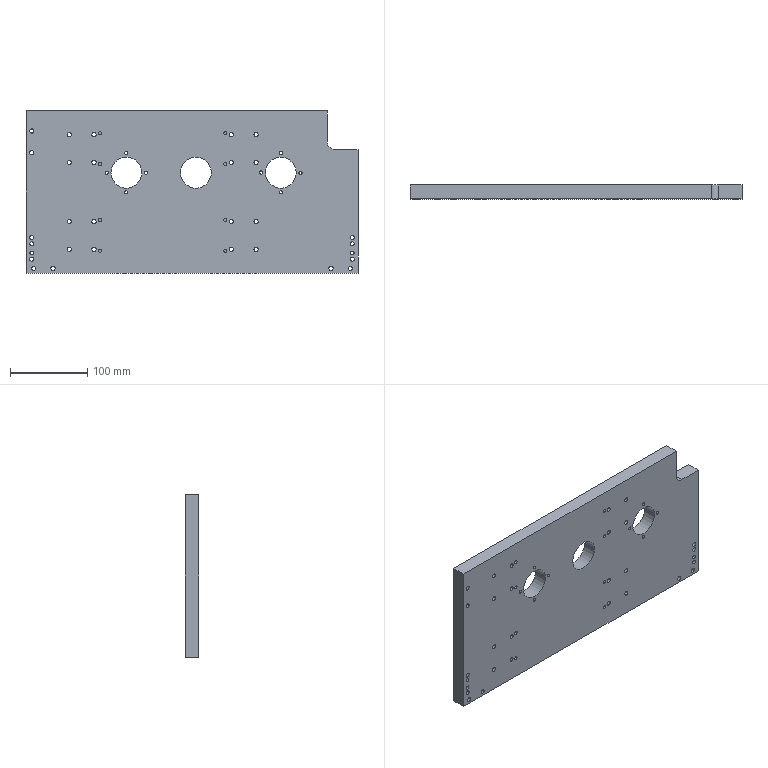Component | SolidWorks | PressingMechanism-06-1 | 1 solid | 193 faces | box 430 x 18 x 210 mm | volume 1498905 mm3 | cylinder 151 | plane 42 | commonest cylinder face diameters 10 x52 5.5 x52 4 x16 4.2 x16 5 x8 40 x6 20 x1
build123d program:
from build123d import *

# Parameters (mm, degrees)
SKETCH1_W                                           = 210
SKETCH1_H                                           = 480
EXTRUDE1_DEPTH                                      = 9
HOLEWZD1_D                                          = 40
MOVE_FACE1_BY                                       = 50
M5_TAPPED_HOLE1_D                                   = 4.2
CBORE_FOR_M5_HEX_SOCKET_HEAD_CAP_SCREW1_D           = 5.5
CBORE_FOR_M5_HEX_SOCKET_HEAD_CAP_SCREW1_CBORE_D     = 10
CBORE_FOR_M5_HEX_SOCKET_HEAD_CAP_SCREW1_CBORE_DEPTH = 5.4
HOLEWZD2_D                                          = 4
HOLEWZD2_DEPTH                                      = 8
CUT_EXTRUDE2_REACH                                  = 264.581
SKETCH14_W                                          = 50
SKETCH14_H                                          = 40
HOLEWZD3_D                                          = 5
CBORE_FOR_M5_HEX_SOCKET_HEAD_CAP_SCREW2_D           = 5.5
CBORE_FOR_M5_HEX_SOCKET_HEAD_CAP_SCREW2_CBORE_D     = 10
CBORE_FOR_M5_HEX_SOCKET_HEAD_CAP_SCREW2_CBORE_DEPTH = 5.4
FILLET1_R                                           = 10


with BuildPart() as part:
    # Sketch1 → Extrude1 (new, symmetric)
    with BuildSketch(Plane(origin=(0, 0, 0), x_dir=(1, 0, 0), z_dir=(0, 1, 0))):
        Rectangle(SKETCH1_W, SKETCH1_H)
    extrude(amount=EXTRUDE1_DEPTH, both=True)

    # HoleWzd1 (through all)
    with Locations(Plane(origin=(0, 9, 0), x_dir=(1, 0, 0), z_dir=(0, 1, 0))):
        with Locations((25, 30), (25, 140), (25, -60)):
            Hole(HOLEWZD1_D / 2)

    # Move Face1: a face moved inward by 50.0
    extrude(part.faces().sort_by_distance((0, 0, 240))[0], amount=MOVE_FACE1_BY, dir=(0, 0, -1), mode=Mode.SUBTRACT)

    # M5 Tapped Hole1 (through all)
    with Locations(Plane(origin=(0, 9, 0), x_dir=(1, 0, 0), z_dir=(0, 1, 0))):
        with Locations((25, -34.5), (-0.5, -60), (25, -85.5), (50.5, -60), (24.785, 165.499), (-0.4991, 139.785), (25.215, 114.501), (50.499, 140.215)):
            Hole(M5_TAPPED_HOLE1_D / 2)

    # CBORE for M5 Hex Socket Head Cap Screw1 (through all)
    with Locations(Plane(origin=(0, 9, 0), x_dir=(1, 0, 0), z_dir=(0, 1, 0))):
        with Locations((74.25, 108), (38.25, 108), (38.25, 76), (74.25, 76), (74.25, -102), (38.25, -102), (38.25, -134), (74.25, -134), (-74.25, -102), (-74.25, -134), (-38.25, -134), (-38.25, -102), (-74.25, 108), (-74.25, 76), (-38.25, 76), (-38.25, 108)):
            CounterBoreHole(CBORE_FOR_M5_HEX_SOCKET_HEAD_CAP_SCREW1_D / 2, CBORE_FOR_M5_HEX_SOCKET_HEAD_CAP_SCREW1_CBORE_D / 2, CBORE_FOR_M5_HEX_SOCKET_HEAD_CAP_SCREW1_CBORE_DEPTH)

    # HoleWzd2
    with Locations(Plane(origin=(0, -9, 0), x_dir=(-1, 0, 0), z_dir=(0, -1, 0))):
        with Locations((-76.25, 68), (-36.25, 68), (36.25, 68), (76.25, 68), (36.25, -94), (76.25, -94), (-76.25, -94), (-36.25, -94)):
            Hole(HOLEWZD2_D / 2, depth=HOLEWZD2_DEPTH)

    # Sketch14 → Cut-Extrude2 (cut, up to next)
    with BuildSketch(Plane(origin=(0, 9, 0), x_dir=(1, 0, 0), z_dir=(0, 1, 0)), mode=Mode.PRIVATE) as cut_extrude2_sk1:
        with Locations((80, 220)):
            Rectangle(SKETCH14_W, SKETCH14_H)
    cut_extrude2_tool1 = extrude(cut_extrude2_sk1.sketch, amount=-CUT_EXTRUDE2_REACH, mode=Mode.PRIVATE) & part.part
    add(cut_extrude2_tool1.solids().sort_by_distance((80, 9, -220))[0], mode=Mode.SUBTRACT)

    # HoleWzd3 (through all)
    with Locations(Plane(origin=(0, 9, 0), x_dir=(1, 0, 0), z_dir=(0, 1, 0))):
        with Locations((-79, -182.5), (-67, -182.5), (-67, 232.5), (-79, 232.5)):
            Hole(HOLEWZD3_D / 2)

    # CBORE for M5 Hex Socket Head Cap Screw2 (through all)
    with Locations(Plane(origin=(0, 9, 0), x_dir=(1, 0, 0), z_dir=(0, 1, 0))):
        with Locations((79, -182.5), (51, -182.5), (-59, -182.5), (-87, -182.5), (-99, -180), (-99, -155), (-99, 230), (-99, 205), (-87, 232.5), (-59, 232.5)):
            CounterBoreHole(CBORE_FOR_M5_HEX_SOCKET_HEAD_CAP_SCREW2_D / 2, CBORE_FOR_M5_HEX_SOCKET_HEAD_CAP_SCREW2_CBORE_D / 2, CBORE_FOR_M5_HEX_SOCKET_HEAD_CAP_SCREW2_CBORE_DEPTH)

    # Fillet1
    fillet1_edges = [part.edges().sort_by_distance(p)[0] for p in [
        (55, 0, -200),
    ]]
    fillet(fillet1_edges, radius=FILLET1_R)


solid = part.part

# Placed as in the assembly
solid = solid.moved(Location((-10, 54, 150), (0, -90, 0)))